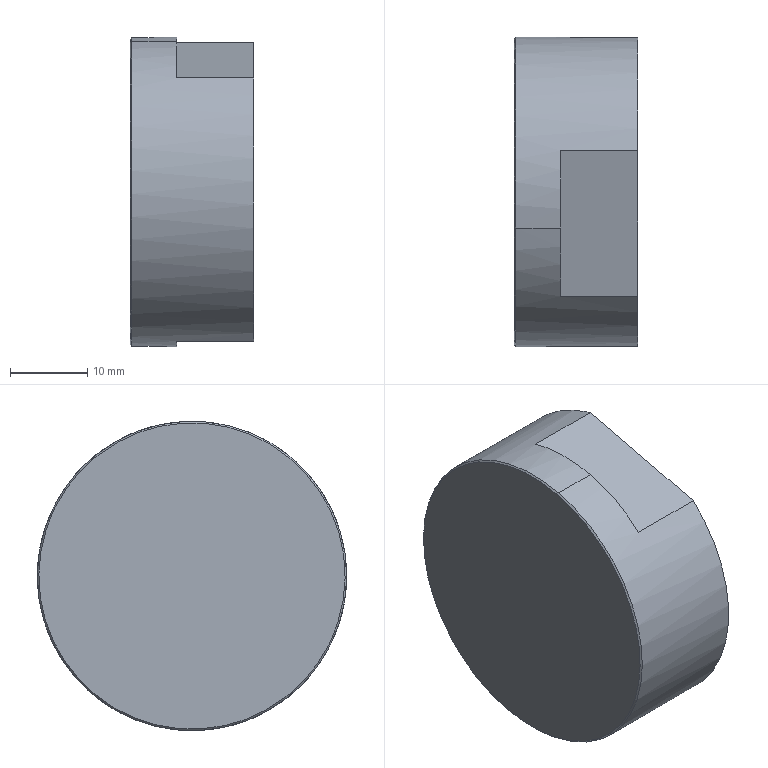Component | SolidWorks | CS021-A10-A008-1 | 1 solid | 14 faces | box 16 x 40 x 40 mm | volume 19065 mm3 | plane 6 | cylinder 4 | cone 4 | commonest cylinder face diameters 6 x2 40 x2 | material SUS304
build123d program:
from build123d import *

# Parameters (mm, degrees)
SKETCH1_R             = 20
BOSS_EXTRUDE1_DEPTH   = 8
CHAMFER1_SIZE         = 0.2
M6_TAPPED_HOLE1_D     = 6
M6_TAPPED_HOLE1_DEPTH = 13
M6_TAPPED_HOLE1_TIP   = 1.803
SKETCH4_OUTSIDE_W     = 53.758
SKETCH4_OUTSIDE_H     = 53.758
SKETCH4_OUTSIDE_W_2   = 35
SKETCH4_OUTSIDE_H_2   = 51.714
CUT_EXTRUDE1_DEPTH    = 10


with BuildPart() as part:
    # Sketch1 → Boss-Extrude1 (new, symmetric)
    with BuildSketch(Plane(origin=(0, 0, 0), x_dir=(0, 0, -1), z_dir=(1, 0, 0))):
        Circle(SKETCH1_R)
    extrude(amount=BOSS_EXTRUDE1_DEPTH, both=True)

    # Chamfer1
    chamfer1_edges = [part.edges().sort_by_distance(p)[0] for p in [
        (-8, 0, 20),
    ]]
    chamfer(chamfer1_edges, length=CHAMFER1_SIZE)

    # M6 Tapped Hole1
    with Locations(Plane(origin=(8, 0, 0), x_dir=(0, 0, -1), z_dir=(1, 0, 0))):
        with Locations((0, 0)):
            Hole(M6_TAPPED_HOLE1_D / 2, depth=M6_TAPPED_HOLE1_DEPTH)
            with Locations((0, 0, -(M6_TAPPED_HOLE1_DEPTH + M6_TAPPED_HOLE1_TIP / 2))):  # 118° drill point
                Cone(0, M6_TAPPED_HOLE1_D / 2, M6_TAPPED_HOLE1_TIP, mode=Mode.SUBTRACT)

    # Sketch4 outside → Cut-Extrude1 (cut)
    with BuildSketch(Plane(origin=(8, 0, 0), x_dir=(0, 0, -1), z_dir=(1, 0, 0))):
        Rectangle(SKETCH4_OUTSIDE_W, SKETCH4_OUTSIDE_H)
        Rectangle(SKETCH4_OUTSIDE_W_2, SKETCH4_OUTSIDE_H_2, mode=Mode.SUBTRACT)
    extrude(amount=-CUT_EXTRUDE1_DEPTH, mode=Mode.SUBTRACT)


solid = part.part

# Placed as in the assembly
solid = solid.moved(Location((19.448, 172.317, 0), (13.563, 0, 0)))
STEP:
#1=COLOUR_RGB('',0.7922,0.8196,0.9333);
#2=FILL_AREA_STYLE_COLOUR('',#1);
#3=FILL_AREA_STYLE('',(#2));
#4=SURFACE_STYLE_FILL_AREA(#3);
#5=SURFACE_SIDE_STYLE('',(#4));
#6=SURFACE_STYLE_USAGE(.BOTH.,#5);
#7=PRESENTATION_STYLE_ASSIGNMENT((#6));
#8=CARTESIAN_POINT('',(0.5688,6.756,0.1148));
#9=VERTEX_POINT('',#8);
#10=CARTESIAN_POINT('',(0.5688,6.812,-0.1148));
#11=VERTEX_POINT('',#10);
#12=CARTESIAN_POINT('',(0.5688,6.784,0.));
#13=DIRECTION('',(1.,0.,0.));
#14=DIRECTION('',(0.,0.2345,-0.9721));
#15=AXIS2_PLACEMENT_3D('',#12,#13,#14);
#16=CIRCLE('',#15,0.1181);
#17=EDGE_CURVE('',#9,#11,#16,.T.);
#18=ORIENTED_EDGE('',*,*,#17,.F.);
#19=CARTESIAN_POINT('',(1.081,6.756,0.1148));
#20=VERTEX_POINT('',#19);
#21=CARTESIAN_POINT('',(1.081,6.756,0.1148));
#22=DIRECTION('',(1.,0.,0.));
#23=VECTOR('',#22,39.37);
#24=LINE('',#21,#23);
#25=EDGE_CURVE('',#9,#20,#24,.T.);
#26=ORIENTED_EDGE('',*,*,#25,.T.);
#27=CARTESIAN_POINT('',(1.081,6.812,-0.1148));
#28=VERTEX_POINT('',#27);
#29=CARTESIAN_POINT('',(1.081,6.784,0.));
#30=DIRECTION('',(1.,0.,0.));
#31=DIRECTION('',(0.,0.2345,-0.9721));
#32=AXIS2_PLACEMENT_3D('',#29,#30,#31);
#33=CIRCLE('',#32,0.1181);
#34=EDGE_CURVE('',#20,#28,#33,.T.);
#35=ORIENTED_EDGE('',*,*,#34,.T.);
#36=CARTESIAN_POINT('',(1.081,6.812,-0.1148));
#37=DIRECTION('',(1.,0.,0.));
#38=VECTOR('',#37,39.37);
#39=LINE('',#36,#38);
#40=EDGE_CURVE('',#11,#28,#39,.T.);
#41=ORIENTED_EDGE('',*,*,#40,.F.);
#42=EDGE_LOOP('',(#18,#26,#35,#41));
#43=FACE_OUTER_BOUND('',#42,.T.);
#44=CARTESIAN_POINT('',(1.081,6.784,0.));
#45=DIRECTION('',(1.,0.,0.));
#46=DIRECTION('',(0.,0.2345,-0.9721));
#47=AXIS2_PLACEMENT_3D('',#44,#45,#46);
#48=CYLINDRICAL_SURFACE('',#47,0.1181);
#49=ADVANCED_FACE('',(#43),#48,.F.);
#50=CARTESIAN_POINT('',(0.4978,6.784,0.));
#51=VERTEX_POINT('',#50);
#52=CARTESIAN_POINT('',(0.5688,6.812,-0.1148));
#53=DIRECTION('',(0.515,0.201,-0.8333));
#54=VECTOR('',#53,39.37);
#55=LINE('',#52,#54);
#56=EDGE_CURVE('',#51,#11,#55,.T.);
#57=ORIENTED_EDGE('',*,*,#56,.F.);
#58=CARTESIAN_POINT('',(0.5688,6.756,0.1148));
#59=DIRECTION('',(0.515,-0.201,0.8333));
#60=VECTOR('',#59,39.37);
#61=LINE('',#58,#60);
#62=EDGE_CURVE('',#51,#9,#61,.T.);
#63=ORIENTED_EDGE('',*,*,#62,.T.);
#64=ORIENTED_EDGE('',*,*,#17,.T.);
#65=EDGE_LOOP('',(#57,#63,#64));
#66=FACE_OUTER_BOUND('',#65,.T.);
#67=CARTESIAN_POINT('',(0.5688,6.784,0.));
#68=DIRECTION('',(1.,0.,0.));
#69=DIRECTION('',(0.,0.2345,-0.9721));
#70=AXIS2_PLACEMENT_3D('',#67,#68,#69);
#71=CONICAL_SURFACE('',#70,0.1181,1.03);
#72=ADVANCED_FACE('',(#66),#71,.F.);
#73=CARTESIAN_POINT('',(0.4507,6.601,0.7578));
#74=VERTEX_POINT('',#73);
#75=CARTESIAN_POINT('',(0.4507,6.967,-0.7578));
#76=VERTEX_POINT('',#75);
#77=CARTESIAN_POINT('',(0.4507,6.784,0.));
#78=DIRECTION('',(-1.,0.,0.));
#79=DIRECTION('',(0.,0.2345,-0.9721));
#80=AXIS2_PLACEMENT_3D('',#77,#78,#79);
#81=CIRCLE('',#80,0.7795);
#82=EDGE_CURVE('',#74,#76,#81,.T.);
#83=ORIENTED_EDGE('',*,*,#82,.F.);
#84=CARTESIAN_POINT('',(0.4586,6.599,0.7654));
#85=VERTEX_POINT('',#84);
#86=CARTESIAN_POINT('',(0.4586,6.599,0.7654));
#87=DIRECTION('',(0.7071,-0.1658,0.6874));
#88=VECTOR('',#87,39.37);
#89=LINE('',#86,#88);
#90=EDGE_CURVE('',#74,#85,#89,.T.);
#91=ORIENTED_EDGE('',*,*,#90,.T.);
#92=CARTESIAN_POINT('',(0.4586,6.969,-0.7654));
#93=VERTEX_POINT('',#92);
#94=CARTESIAN_POINT('',(0.4586,6.784,0.));
#95=DIRECTION('',(1.,0.,0.));
#96=DIRECTION('',(0.,0.2345,-0.9721));
#97=AXIS2_PLACEMENT_3D('',#94,#95,#96);
#98=CIRCLE('',#97,0.7874);
#99=EDGE_CURVE('',#93,#85,#98,.T.);
#100=ORIENTED_EDGE('',*,*,#99,.F.);
#101=CARTESIAN_POINT('',(0.4586,6.969,-0.7654));
#102=DIRECTION('',(0.7071,0.1658,-0.6874));
#103=VECTOR('',#102,39.37);
#104=LINE('',#101,#103);
#105=EDGE_CURVE('',#76,#93,#104,.T.);
#106=ORIENTED_EDGE('',*,*,#105,.F.);
#107=EDGE_LOOP('',(#83,#91,#100,#106));
#108=FACE_OUTER_BOUND('',#107,.T.);
#109=CARTESIAN_POINT('',(0.4586,6.784,0.));
#110=DIRECTION('',(1.,0.,0.));
#111=DIRECTION('',(0.,0.2345,-0.9721));
#112=AXIS2_PLACEMENT_3D('',#109,#110,#111);
#113=CONICAL_SURFACE('',#112,0.7874,0.7854);
#114=ADVANCED_FACE('',(#108),#113,.T.);
#115=CARTESIAN_POINT('',(0.6869,6.969,-0.7654));
#116=VERTEX_POINT('',#115);
#117=CARTESIAN_POINT('',(0.6869,7.316,-0.5804));
#118=VERTEX_POINT('',#117);
#119=CARTESIAN_POINT('',(0.6869,6.784,0.));
#120=DIRECTION('',(1.,0.,0.));
#121=DIRECTION('',(0.,0.2345,-0.9721));
#122=AXIS2_PLACEMENT_3D('',#119,#120,#121);
#123=CIRCLE('',#122,0.7874);
#124=EDGE_CURVE('',#116,#118,#123,.T.);
#125=ORIENTED_EDGE('',*,*,#124,.F.);
#126=CARTESIAN_POINT('',(1.081,6.969,-0.7654));
#127=DIRECTION('',(-1.,0.,0.));
#128=VECTOR('',#127,39.37);
#129=LINE('',#126,#128);
#130=EDGE_CURVE('',#116,#93,#129,.T.);
#131=ORIENTED_EDGE('',*,*,#130,.T.);
#132=ORIENTED_EDGE('',*,*,#99,.T.);
#133=CARTESIAN_POINT('',(0.6869,6.599,0.7654));
#134=VERTEX_POINT('',#133);
#135=CARTESIAN_POINT('',(1.081,6.599,0.7654));
#136=DIRECTION('',(-1.,0.,0.));
#137=VECTOR('',#136,39.37);
#138=LINE('',#135,#137);
#139=EDGE_CURVE('',#134,#85,#138,.T.);
#140=ORIENTED_EDGE('',*,*,#139,.F.);
#141=CARTESIAN_POINT('',(0.6869,6.993,0.7592));
#142=VERTEX_POINT('',#141);
#143=CARTESIAN_POINT('',(0.6869,6.784,0.));
#144=DIRECTION('',(1.,0.,0.));
#145=DIRECTION('',(0.,0.2345,-0.9721));
#146=AXIS2_PLACEMENT_3D('',#143,#144,#145);
#147=CIRCLE('',#146,0.7874);
#148=EDGE_CURVE('',#142,#134,#147,.T.);
#149=ORIENTED_EDGE('',*,*,#148,.F.);
#150=CARTESIAN_POINT('',(1.081,6.993,0.7592));
#151=VERTEX_POINT('',#150);
#152=CARTESIAN_POINT('',(1.081,6.993,0.7592));
#153=DIRECTION('',(-1.,0.,0.));
#154=VECTOR('',#153,39.37);
#155=LINE('',#152,#154);
#156=EDGE_CURVE('',#151,#142,#155,.T.);
#157=ORIENTED_EDGE('',*,*,#156,.F.);
#158=CARTESIAN_POINT('',(1.081,7.316,-0.5804));
#159=VERTEX_POINT('',#158);
#160=CARTESIAN_POINT('',(1.081,6.784,0.));
#161=DIRECTION('',(1.,0.,0.));
#162=DIRECTION('',(0.,0.2345,-0.9721));
#163=AXIS2_PLACEMENT_3D('',#160,#161,#162);
#164=CIRCLE('',#163,0.7874);
#165=EDGE_CURVE('',#159,#151,#164,.T.);
#166=ORIENTED_EDGE('',*,*,#165,.F.);
#167=CARTESIAN_POINT('',(1.081,7.316,-0.5804));
#168=DIRECTION('',(1.,0.,0.));
#169=VECTOR('',#168,39.37);
#170=LINE('',#167,#169);
#171=EDGE_CURVE('',#118,#159,#170,.T.);
#172=ORIENTED_EDGE('',*,*,#171,.F.);
#173=EDGE_LOOP('',(#125,#131,#132,#140,#149,#157,#166,#172));
#174=FACE_OUTER_BOUND('',#173,.T.);
#175=CARTESIAN_POINT('',(1.081,6.784,0.));
#176=DIRECTION('',(-1.,0.,0.));
#177=DIRECTION('',(0.,-0.2345,0.9721));
#178=AXIS2_PLACEMENT_3D('',#175,#176,#177);
#179=CYLINDRICAL_SURFACE('',#178,0.7874);
#180=ADVANCED_FACE('',(#174),#179,.T.);
#181=ORIENTED_EDGE('',*,*,#130,.F.);
#182=CARTESIAN_POINT('',(0.6869,6.575,-0.7592));
#183=VERTEX_POINT('',#182);
#184=CARTESIAN_POINT('',(0.6869,6.784,0.));
#185=DIRECTION('',(1.,0.,0.));
#186=DIRECTION('',(0.,0.2345,-0.9721));
#187=AXIS2_PLACEMENT_3D('',#184,#185,#186);
#188=CIRCLE('',#187,0.7874);
#189=EDGE_CURVE('',#183,#116,#188,.T.);
#190=ORIENTED_EDGE('',*,*,#189,.F.);
#191=CARTESIAN_POINT('',(1.081,6.575,-0.7592));
#192=VERTEX_POINT('',#191);
#193=CARTESIAN_POINT('',(1.081,6.575,-0.7592));
#194=DIRECTION('',(-1.,0.,0.));
#195=VECTOR('',#194,39.37);
#196=LINE('',#193,#195);
#197=EDGE_CURVE('',#192,#183,#196,.T.);
#198=ORIENTED_EDGE('',*,*,#197,.F.);
#199=CARTESIAN_POINT('',(1.081,6.252,0.5804));
#200=VERTEX_POINT('',#199);
#201=CARTESIAN_POINT('',(1.081,6.784,0.));
#202=DIRECTION('',(1.,0.,0.));
#203=DIRECTION('',(0.,0.2345,-0.9721));
#204=AXIS2_PLACEMENT_3D('',#201,#202,#203);
#205=CIRCLE('',#204,0.7874);
#206=EDGE_CURVE('',#200,#192,#205,.T.);
#207=ORIENTED_EDGE('',*,*,#206,.F.);
#208=CARTESIAN_POINT('',(0.6869,6.252,0.5804));
#209=VERTEX_POINT('',#208);
#210=CARTESIAN_POINT('',(1.081,6.252,0.5804));
#211=DIRECTION('',(1.,0.,0.));
#212=VECTOR('',#211,39.37);
#213=LINE('',#210,#212);
#214=EDGE_CURVE('',#209,#200,#213,.T.);
#215=ORIENTED_EDGE('',*,*,#214,.F.);
#216=CARTESIAN_POINT('',(0.6869,6.784,0.));
#217=DIRECTION('',(1.,0.,0.));
#218=DIRECTION('',(0.,0.2345,-0.9721));
#219=AXIS2_PLACEMENT_3D('',#216,#217,#218);
#220=CIRCLE('',#219,0.7874);
#221=EDGE_CURVE('',#134,#209,#220,.T.);
#222=ORIENTED_EDGE('',*,*,#221,.F.);
#223=ORIENTED_EDGE('',*,*,#139,.T.);
#224=CARTESIAN_POINT('',(0.4586,6.784,0.));
#225=DIRECTION('',(1.,0.,0.));
#226=DIRECTION('',(0.,0.2345,-0.9721));
#227=AXIS2_PLACEMENT_3D('',#224,#225,#226);
#228=CIRCLE('',#227,0.7874);
#229=EDGE_CURVE('',#85,#93,#228,.T.);
#230=ORIENTED_EDGE('',*,*,#229,.T.);
#231=EDGE_LOOP('',(#181,#190,#198,#207,#215,#222,#223,#230));
#232=FACE_OUTER_BOUND('',#231,.T.);
#233=CARTESIAN_POINT('',(1.081,6.784,0.));
#234=DIRECTION('',(-1.,0.,0.));
#235=DIRECTION('',(0.,-0.2345,0.9721));
#236=AXIS2_PLACEMENT_3D('',#233,#234,#235);
#237=CYLINDRICAL_SURFACE('',#236,0.7874);
#238=ADVANCED_FACE('',(#232),#237,.T.);
#239=CARTESIAN_POINT('',(1.081,6.784,0.));
#240=DIRECTION('',(1.,0.,0.));
#241=DIRECTION('',(0.,0.2345,-0.9721));
#242=AXIS2_PLACEMENT_3D('',#239,#240,#241);
#243=CIRCLE('',#242,0.1181);
#244=EDGE_CURVE('',#28,#20,#243,.T.);
#245=ORIENTED_EDGE('',*,*,#244,.F.);
#246=ORIENTED_EDGE('',*,*,#34,.F.);
#247=EDGE_LOOP('',(#245,#246));
#248=FACE_BOUND('',#247,.T.);
#249=ORIENTED_EDGE('',*,*,#206,.T.);
#250=CARTESIAN_POINT('',(1.081,6.946,-0.6698));
#251=DIRECTION('',(0.,0.9721,0.2345));
#252=VECTOR('',#251,39.37);
#253=LINE('',#250,#252);
#254=EDGE_CURVE('',#192,#159,#253,.T.);
#255=ORIENTED_EDGE('',*,*,#254,.T.);
#256=ORIENTED_EDGE('',*,*,#165,.T.);
#257=CARTESIAN_POINT('',(1.081,6.623,0.6698));
#258=DIRECTION('',(0.,-0.9721,-0.2345));
#259=VECTOR('',#258,39.37);
#260=LINE('',#257,#259);
#261=EDGE_CURVE('',#151,#200,#260,.T.);
#262=ORIENTED_EDGE('',*,*,#261,.T.);
#263=EDGE_LOOP('',(#249,#255,#256,#262));
#264=FACE_OUTER_BOUND('',#263,.T.);
#265=CARTESIAN_POINT('',(1.081,6.784,0.));
#266=DIRECTION('',(1.,0.,0.));
#267=DIRECTION('',(0.,0.2345,-0.9721));
#268=AXIS2_PLACEMENT_3D('',#265,#266,#267);
#269=PLANE('',#268);
#270=ADVANCED_FACE('',(#248,#264),#269,.T.);
#271=CARTESIAN_POINT('',(0.4507,6.784,0.));
#272=DIRECTION('',(-1.,0.,0.));
#273=DIRECTION('',(0.,0.2345,-0.9721));
#274=AXIS2_PLACEMENT_3D('',#271,#272,#273);
#275=CIRCLE('',#274,0.7795);
#276=EDGE_CURVE('',#76,#74,#275,.T.);
#277=ORIENTED_EDGE('',*,*,#276,.T.);
#278=ORIENTED_EDGE('',*,*,#82,.T.);
#279=EDGE_LOOP('',(#277,#278));
#280=FACE_OUTER_BOUND('',#279,.T.);
#281=CARTESIAN_POINT('',(0.4507,6.784,0.));
#282=DIRECTION('',(1.,0.,0.));
#283=DIRECTION('',(0.,0.2345,-0.9721));
#284=AXIS2_PLACEMENT_3D('',#281,#282,#283);
#285=PLANE('',#284);
#286=ADVANCED_FACE('',(#280),#285,.F.);
#287=ORIENTED_EDGE('',*,*,#90,.F.);
#288=ORIENTED_EDGE('',*,*,#276,.F.);
#289=ORIENTED_EDGE('',*,*,#105,.T.);
#290=ORIENTED_EDGE('',*,*,#229,.F.);
#291=EDGE_LOOP('',(#287,#288,#289,#290));
#292=FACE_OUTER_BOUND('',#291,.T.);
#293=CARTESIAN_POINT('',(0.4586,6.784,0.));
#294=DIRECTION('',(1.,0.,0.));
#295=DIRECTION('',(0.,0.2345,-0.9721));
#296=AXIS2_PLACEMENT_3D('',#293,#294,#295);
#297=CONICAL_SURFACE('',#296,0.7874,0.7854);
#298=ADVANCED_FACE('',(#292),#297,.T.);
#299=ORIENTED_EDGE('',*,*,#62,.F.);
#300=ORIENTED_EDGE('',*,*,#56,.T.);
#301=CARTESIAN_POINT('',(0.5688,6.784,0.));
#302=DIRECTION('',(1.,0.,0.));
#303=DIRECTION('',(0.,0.2345,-0.9721));
#304=AXIS2_PLACEMENT_3D('',#301,#302,#303);
#305=CIRCLE('',#304,0.1181);
#306=EDGE_CURVE('',#11,#9,#305,.T.);
#307=ORIENTED_EDGE('',*,*,#306,.T.);
#308=EDGE_LOOP('',(#299,#300,#307));
#309=FACE_OUTER_BOUND('',#308,.T.);
#310=CARTESIAN_POINT('',(0.5688,6.784,0.));
#311=DIRECTION('',(1.,0.,0.));
#312=DIRECTION('',(0.,0.2345,-0.9721));
#313=AXIS2_PLACEMENT_3D('',#310,#311,#312);
#314=CONICAL_SURFACE('',#313,0.1181,1.03);
#315=ADVANCED_FACE('',(#309),#314,.F.);
#316=ORIENTED_EDGE('',*,*,#25,.F.);
#317=ORIENTED_EDGE('',*,*,#306,.F.);
#318=ORIENTED_EDGE('',*,*,#40,.T.);
#319=ORIENTED_EDGE('',*,*,#244,.T.);
#320=EDGE_LOOP('',(#316,#317,#318,#319));
#321=FACE_OUTER_BOUND('',#320,.T.);
#322=CARTESIAN_POINT('',(1.081,6.784,0.));
#323=DIRECTION('',(1.,0.,0.));
#324=DIRECTION('',(0.,0.2345,-0.9721));
#325=AXIS2_PLACEMENT_3D('',#322,#323,#324);
#326=CYLINDRICAL_SURFACE('',#325,0.1181);
#327=ADVANCED_FACE('',(#321),#326,.F.);
#328=ORIENTED_EDGE('',*,*,#156,.T.);
#329=CARTESIAN_POINT('',(0.6869,5.633,0.431));
#330=DIRECTION('',(0.,-0.9721,-0.2345));
#331=VECTOR('',#330,39.37);
#332=LINE('',#329,#331);
#333=EDGE_CURVE('',#142,#209,#332,.T.);
#334=ORIENTED_EDGE('',*,*,#333,.T.);
#335=ORIENTED_EDGE('',*,*,#214,.T.);
#336=ORIENTED_EDGE('',*,*,#261,.F.);
#337=EDGE_LOOP('',(#328,#334,#335,#336));
#338=FACE_OUTER_BOUND('',#337,.T.);
#339=CARTESIAN_POINT('',(0.6869,5.633,0.431));
#340=DIRECTION('',(0.,-0.2345,0.9721));
#341=DIRECTION('',(1.,0.,0.));
#342=AXIS2_PLACEMENT_3D('',#339,#340,#341);
#343=PLANE('',#342);
#344=ADVANCED_FACE('',(#338),#343,.T.);
#345=ORIENTED_EDGE('',*,*,#148,.T.);
#346=ORIENTED_EDGE('',*,*,#221,.T.);
#347=ORIENTED_EDGE('',*,*,#333,.F.);
#348=EDGE_LOOP('',(#345,#346,#347));
#349=FACE_OUTER_BOUND('',#348,.T.);
#350=CARTESIAN_POINT('',(0.6869,6.784,0.));
#351=DIRECTION('',(1.,0.,0.));
#352=DIRECTION('',(0.,0.2345,-0.9721));
#353=AXIS2_PLACEMENT_3D('',#350,#351,#352);
#354=PLANE('',#353);
#355=ADVANCED_FACE('',(#349),#354,.T.);
#356=ORIENTED_EDGE('',*,*,#189,.T.);
#357=ORIENTED_EDGE('',*,*,#124,.T.);
#358=CARTESIAN_POINT('',(0.6869,5.956,-0.9085));
#359=DIRECTION('',(0.,0.9721,0.2345));
#360=VECTOR('',#359,39.37);
#361=LINE('',#358,#360);
#362=EDGE_CURVE('',#183,#118,#361,.T.);
#363=ORIENTED_EDGE('',*,*,#362,.F.);
#364=EDGE_LOOP('',(#356,#357,#363));
#365=FACE_OUTER_BOUND('',#364,.T.);
#366=CARTESIAN_POINT('',(0.6869,6.784,0.));
#367=DIRECTION('',(1.,0.,0.));
#368=DIRECTION('',(0.,0.2345,-0.9721));
#369=AXIS2_PLACEMENT_3D('',#366,#367,#368);
#370=PLANE('',#369);
#371=ADVANCED_FACE('',(#365),#370,.T.);
#372=ORIENTED_EDGE('',*,*,#197,.T.);
#373=ORIENTED_EDGE('',*,*,#362,.T.);
#374=ORIENTED_EDGE('',*,*,#171,.T.);
#375=ORIENTED_EDGE('',*,*,#254,.F.);
#376=EDGE_LOOP('',(#372,#373,#374,#375));
#377=FACE_OUTER_BOUND('',#376,.T.);
#378=CARTESIAN_POINT('',(0.6869,5.956,-0.9085));
#379=DIRECTION('',(0.,0.2345,-0.9721));
#380=DIRECTION('',(-1.,0.,0.));
#381=AXIS2_PLACEMENT_3D('',#378,#379,#380);
#382=PLANE('',#381);
#383=ADVANCED_FACE('',(#377),#382,.T.);
#384=CLOSED_SHELL('',(#49,#72,#114,#180,#238,#270,#286,#298,#315,#327,#344,#355,#371,#383));
#385=MANIFOLD_SOLID_BREP('',#384);
#386=STYLED_ITEM('',(#7),#385);
#387=(LENGTH_UNIT()NAMED_UNIT(*)SI_UNIT($,.METRE.));
#388=LENGTH_MEASURE_WITH_UNIT(LENGTH_MEASURE(0.0254),#387);
#389=DIMENSIONAL_EXPONENTS(1.,0.,0.,0.,0.,0.,0.);
#390=(CONVERSION_BASED_UNIT('',#388)LENGTH_UNIT()NAMED_UNIT(#389));
#391=UNCERTAINTY_MEASURE_WITH_UNIT(LENGTH_MEASURE(0.00001),#390,'','');
#392=(NAMED_UNIT(*)PLANE_ANGLE_UNIT()SI_UNIT($,.RADIAN.));
#393=(NAMED_UNIT(*)SI_UNIT($,.STERADIAN.)SOLID_ANGLE_UNIT());
#394=(GEOMETRIC_REPRESENTATION_CONTEXT(3)GLOBAL_UNCERTAINTY_ASSIGNED_CONTEXT((#391))GLOBAL_UNIT_ASSIGNED_CONTEXT((#390,#392,#393))REPRESENTATION_CONTEXT('',''));
#395=MECHANICAL_DESIGN_GEOMETRIC_PRESENTATION_REPRESENTATION('',(#386),#394);
#396=PRESENTATION_LAYER_ASSIGNMENT('','',(#386));
#397=CARTESIAN_POINT('',(0.,0.,0.));
#398=DIRECTION('',(0.,0.,1.));
#399=DIRECTION('',(1.,0.,0.));
#400=AXIS2_PLACEMENT_3D('',#397,#398,#399);
#401=(LENGTH_UNIT()NAMED_UNIT(*)SI_UNIT($,.METRE.));
#402=LENGTH_MEASURE_WITH_UNIT(LENGTH_MEASURE(0.0254),#401);
#403=DIMENSIONAL_EXPONENTS(1.,0.,0.,0.,0.,0.,0.);
#404=(CONVERSION_BASED_UNIT('',#402)LENGTH_UNIT()NAMED_UNIT(#403));
#405=UNCERTAINTY_MEASURE_WITH_UNIT(LENGTH_MEASURE(0.00001),#404,'','');
#406=(NAMED_UNIT(*)PLANE_ANGLE_UNIT()SI_UNIT($,.RADIAN.));
#407=(NAMED_UNIT(*)SI_UNIT($,.STERADIAN.)SOLID_ANGLE_UNIT());
#408=(GEOMETRIC_REPRESENTATION_CONTEXT(3)GLOBAL_UNCERTAINTY_ASSIGNED_CONTEXT((#405))GLOBAL_UNIT_ASSIGNED_CONTEXT((#404,#406,#407))REPRESENTATION_CONTEXT('',''));
#409=ADVANCED_BREP_SHAPE_REPRESENTATION('',(#385,#400),#408);